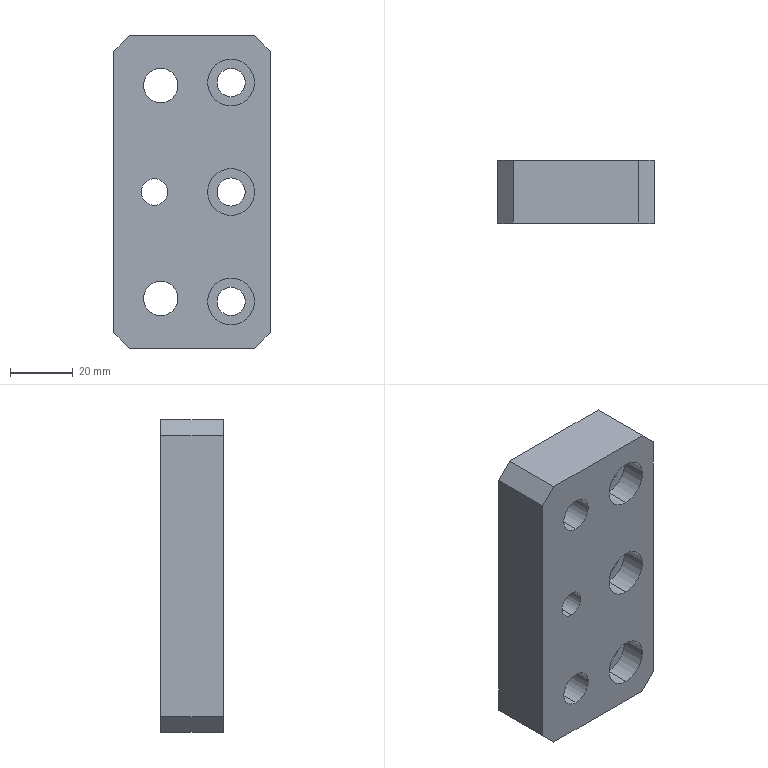Component | SolidWorks | F5-1 | 1 solid | 31 faces | box 50 x 20 x 100 mm | volume 87532 mm3 | cylinder 18 | plane 13 | commonest cylinder face diameters 15 x6 9 x6 11 x4 8.5 x2
build123d program:
from build123d import *

# Parameters (mm, degrees)
SKETCH1_W                                       = 100
SKETCH1_H                                       = 50
BOSS_EXTRUDE1_DEPTH                             = 20
M8_HEX_SOCKET_HEAD_CAP_SCREW_CBORE1_D           = 9
M8_HEX_SOCKET_HEAD_CAP_SCREW_CBORE1_CBORE_D     = 15
M8_HEX_SOCKET_HEAD_CAP_SCREW_CBORE1_CBORE_DEPTH = 8
SKETCH5_R                                       = 5.5
CUT_EXTRUDE1_DEPTH                              = 113.849
M10_TAPPED_HOLE1_D                              = 8.5
CHAMFER1_SIZE                                   = 5


with BuildPart() as part:
    # Sketch1 → Boss-Extrude1 (new body)
    with BuildSketch(Plane.XY):
        with Locations((58.212, 0)):
            Rectangle(SKETCH1_W, SKETCH1_H)
    extrude(amount=BOSS_EXTRUDE1_DEPTH)

    # M8 Hex Socket Head Cap Screw CBORE1 (through all)
    with Locations(Plane.XY.offset(20)):
        with Locations((58.212, 12.5), (23.212, 12.5), (93.212, 12.5)):
            CounterBoreHole(M8_HEX_SOCKET_HEAD_CAP_SCREW_CBORE1_D / 2, M8_HEX_SOCKET_HEAD_CAP_SCREW_CBORE1_CBORE_D / 2, M8_HEX_SOCKET_HEAD_CAP_SCREW_CBORE1_CBORE_DEPTH)

    # Sketch5 → Cut-Extrude1 (cut, through all)
    with BuildSketch(Plane.XY.offset(20)):
        with Locations((24.212, -10)):
            Circle(SKETCH5_R)
        with Locations((92.212, -10)):
            Circle(SKETCH5_R)
    extrude(amount=-CUT_EXTRUDE1_DEPTH, mode=Mode.SUBTRACT)

    # M10 Tapped Hole1 (through all)
    with Locations(Plane.XY.offset(20)):
        with Locations((58.212, -12)):
            Hole(M10_TAPPED_HOLE1_D / 2)

    # Chamfer1
    chamfer1_edges = [part.edges().sort_by_distance(p)[0] for p in [
        (8.212, 25, 10),
        (108.212, 25, 10),
        (108.212, -25, 10),
        (8.212, -25, 10),
    ]]
    chamfer(chamfer1_edges, length=CHAMFER1_SIZE)


solid = part.part

# Placed as in the assembly
solid = solid.moved(Location((96, -206.721, 2.212), (90, 0, -90)))